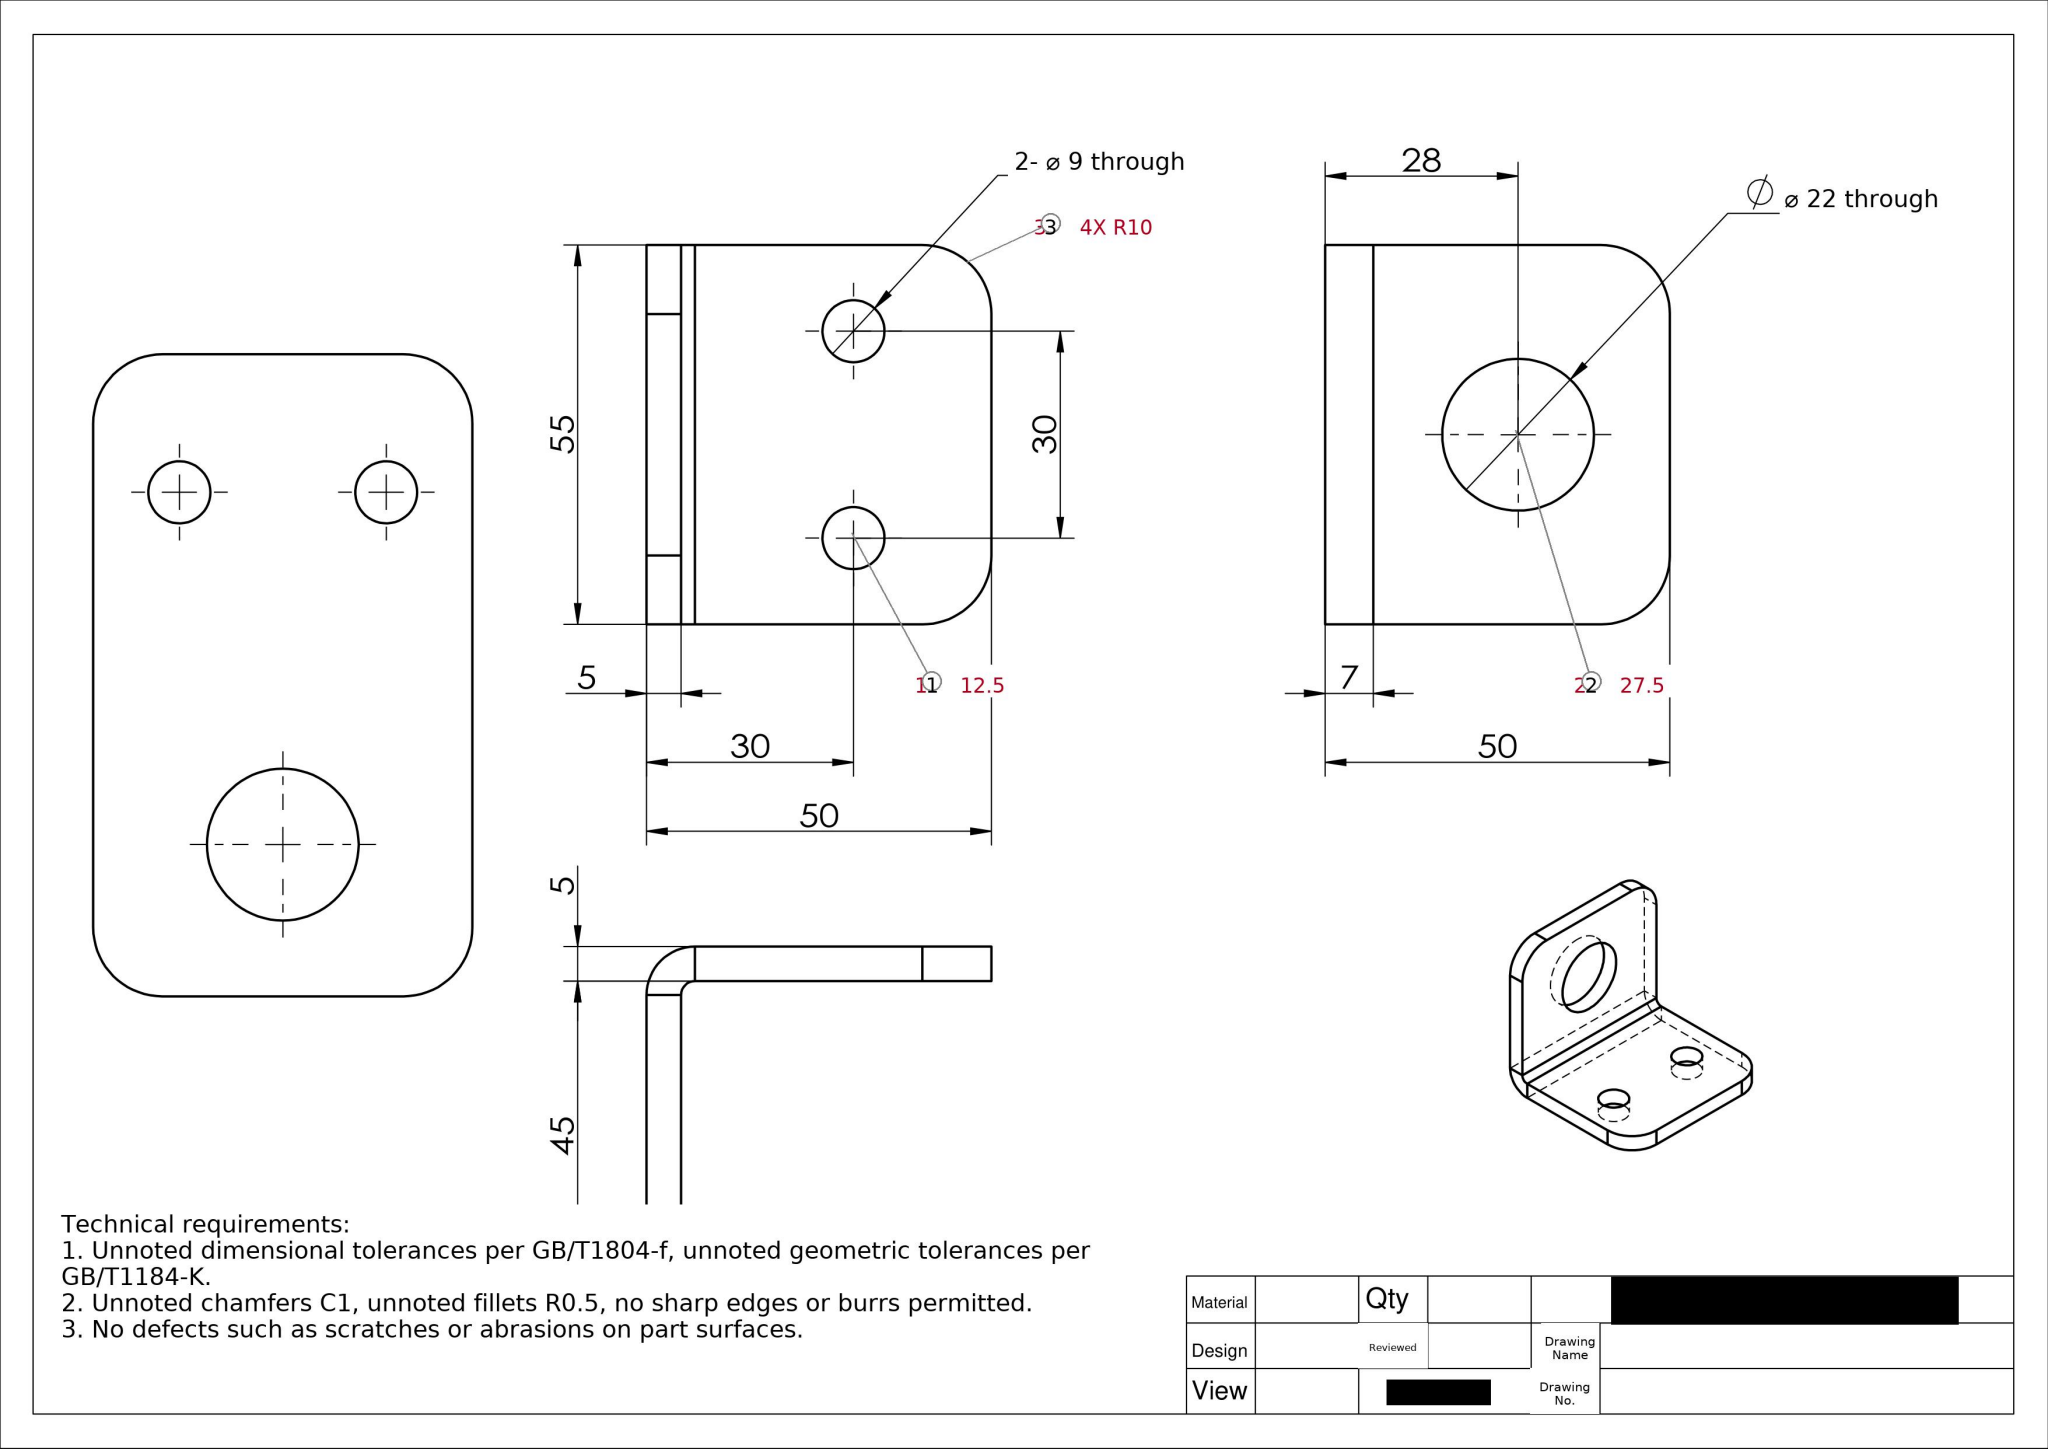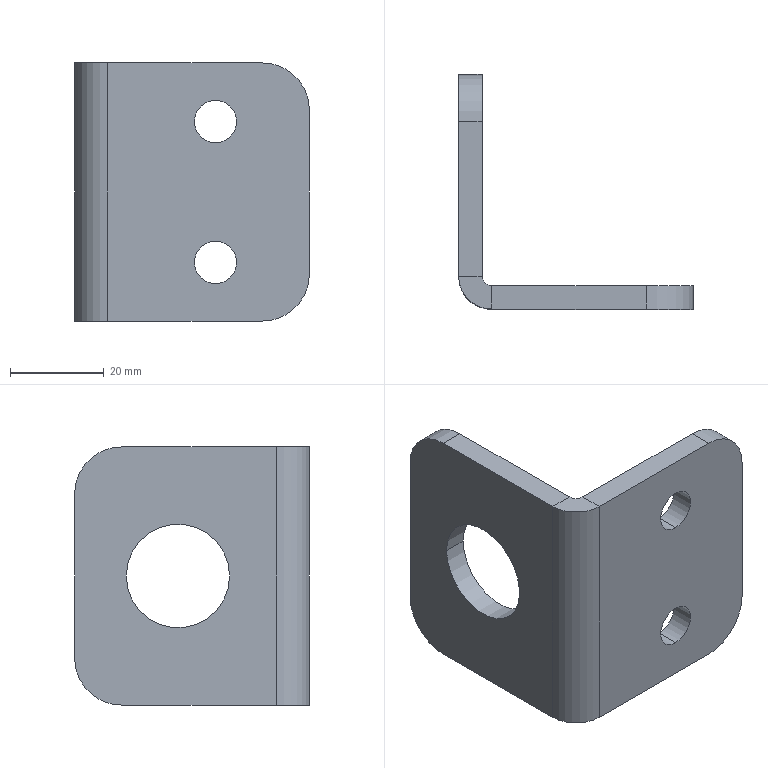Part | SolidWorks | mm | 1 solid | 24 faces | box 50 x 50 x 55 mm | volume 22628 mm3 | cylinder 12 | plane 12 | commonest cylinder face diameters 9 x4 20 x4 22 x2 4 x1 14 x1
STEP:
#1=CARTESIAN_POINT('',(30.,5.,38.));
#2=VERTEX_POINT('',#1);
#3=CARTESIAN_POINT('',(30.,5.,47.));
#4=VERTEX_POINT('',#3);
#5=CARTESIAN_POINT('',(30.,5.,42.5));
#6=DIRECTION('',(0.,1.,0.));
#7=DIRECTION('',(0.,0.,1.));
#8=AXIS2_PLACEMENT_3D('',#5,#6,#7);
#9=CIRCLE('',#8,4.5);
#10=EDGE_CURVE('',#2,#4,#9,.T.);
#11=ORIENTED_EDGE('',*,*,#10,.T.);
#12=CARTESIAN_POINT('',(30.,0.,47.));
#13=VERTEX_POINT('',#12);
#14=CARTESIAN_POINT('',(30.,10.,47.));
#15=DIRECTION('',(0.,-1.,0.));
#16=VECTOR('',#15,1000.);
#17=LINE('',#14,#16);
#18=EDGE_CURVE('',#4,#13,#17,.T.);
#19=ORIENTED_EDGE('',*,*,#18,.T.);
#20=CARTESIAN_POINT('',(30.,0.,38.));
#21=VERTEX_POINT('',#20);
#22=CARTESIAN_POINT('',(30.,0.,42.5));
#23=DIRECTION('',(0.,-1.,0.));
#24=DIRECTION('',(0.,0.,-1.));
#25=AXIS2_PLACEMENT_3D('',#22,#23,#24);
#26=CIRCLE('',#25,4.5);
#27=EDGE_CURVE('',#13,#21,#26,.T.);
#28=ORIENTED_EDGE('',*,*,#27,.T.);
#29=CARTESIAN_POINT('',(30.,10.,38.));
#30=DIRECTION('',(0.,-1.,0.));
#31=VECTOR('',#30,1000.);
#32=LINE('',#29,#31);
#33=EDGE_CURVE('',#2,#21,#32,.T.);
#34=ORIENTED_EDGE('',*,*,#33,.F.);
#35=EDGE_LOOP('',(#11,#19,#28,#34));
#36=FACE_OUTER_BOUND('',#35,.T.);
#37=CARTESIAN_POINT('',(30.,10.,42.5));
#38=DIRECTION('',(0.,-1.,0.));
#39=DIRECTION('',(0.,0.,-1.));
#40=AXIS2_PLACEMENT_3D('',#37,#38,#39);
#41=CYLINDRICAL_SURFACE('',#40,4.5);
#42=ADVANCED_FACE('',(#36),#41,.F.);
#43=CARTESIAN_POINT('',(30.,5.,8.));
#44=VERTEX_POINT('',#43);
#45=CARTESIAN_POINT('',(30.,5.,17.));
#46=VERTEX_POINT('',#45);
#47=CARTESIAN_POINT('',(30.,5.,12.5));
#48=DIRECTION('',(0.,1.,0.));
#49=DIRECTION('',(0.,0.,1.));
#50=AXIS2_PLACEMENT_3D('',#47,#48,#49);
#51=CIRCLE('',#50,4.5);
#52=EDGE_CURVE('',#44,#46,#51,.T.);
#53=ORIENTED_EDGE('',*,*,#52,.T.);
#54=CARTESIAN_POINT('',(30.,0.,17.));
#55=VERTEX_POINT('',#54);
#56=CARTESIAN_POINT('',(30.,10.,17.));
#57=DIRECTION('',(0.,-1.,0.));
#58=VECTOR('',#57,1000.);
#59=LINE('',#56,#58);
#60=EDGE_CURVE('',#46,#55,#59,.T.);
#61=ORIENTED_EDGE('',*,*,#60,.T.);
#62=CARTESIAN_POINT('',(30.,0.,8.));
#63=VERTEX_POINT('',#62);
#64=CARTESIAN_POINT('',(30.,0.,12.5));
#65=DIRECTION('',(0.,-1.,0.));
#66=DIRECTION('',(0.,0.,-1.));
#67=AXIS2_PLACEMENT_3D('',#64,#65,#66);
#68=CIRCLE('',#67,4.5);
#69=EDGE_CURVE('',#55,#63,#68,.T.);
#70=ORIENTED_EDGE('',*,*,#69,.T.);
#71=CARTESIAN_POINT('',(30.,10.,8.));
#72=DIRECTION('',(0.,-1.,0.));
#73=VECTOR('',#72,1000.);
#74=LINE('',#71,#73);
#75=EDGE_CURVE('',#44,#63,#74,.T.);
#76=ORIENTED_EDGE('',*,*,#75,.F.);
#77=EDGE_LOOP('',(#53,#61,#70,#76));
#78=FACE_OUTER_BOUND('',#77,.T.);
#79=CARTESIAN_POINT('',(30.,10.,12.5));
#80=DIRECTION('',(0.,-1.,0.));
#81=DIRECTION('',(0.,0.,-1.));
#82=AXIS2_PLACEMENT_3D('',#79,#80,#81);
#83=CYLINDRICAL_SURFACE('',#82,4.5);
#84=ADVANCED_FACE('',(#78),#83,.F.);
#85=CARTESIAN_POINT('',(0.,17.,27.5));
#86=VERTEX_POINT('',#85);
#87=CARTESIAN_POINT('',(0.,39.,27.5));
#88=VERTEX_POINT('',#87);
#89=CARTESIAN_POINT('',(0.,28.,27.5));
#90=DIRECTION('',(1.,-0.,0.));
#91=DIRECTION('',(0.,1.,0.));
#92=AXIS2_PLACEMENT_3D('',#89,#90,#91);
#93=CIRCLE('',#92,11.);
#94=EDGE_CURVE('',#86,#88,#93,.T.);
#95=ORIENTED_EDGE('',*,*,#94,.F.);
#96=CARTESIAN_POINT('',(5.,17.,27.5));
#97=VERTEX_POINT('',#96);
#98=CARTESIAN_POINT('',(5.,17.,27.5));
#99=DIRECTION('',(1.,-0.,0.));
#100=VECTOR('',#99,1000.);
#101=LINE('',#98,#100);
#102=EDGE_CURVE('',#86,#97,#101,.T.);
#103=ORIENTED_EDGE('',*,*,#102,.T.);
#104=CARTESIAN_POINT('',(5.,39.,27.5));
#105=VERTEX_POINT('',#104);
#106=CARTESIAN_POINT('',(5.,28.,27.5));
#107=DIRECTION('',(1.,-0.,0.));
#108=DIRECTION('',(0.,1.,0.));
#109=AXIS2_PLACEMENT_3D('',#106,#107,#108);
#110=CIRCLE('',#109,11.);
#111=EDGE_CURVE('',#97,#105,#110,.T.);
#112=ORIENTED_EDGE('',*,*,#111,.T.);
#113=CARTESIAN_POINT('',(5.,39.,27.5));
#114=DIRECTION('',(1.,-0.,0.));
#115=VECTOR('',#114,1000.);
#116=LINE('',#113,#115);
#117=EDGE_CURVE('',#88,#105,#116,.T.);
#118=ORIENTED_EDGE('',*,*,#117,.F.);
#119=EDGE_LOOP('',(#95,#103,#112,#118));
#120=FACE_OUTER_BOUND('',#119,.T.);
#121=CARTESIAN_POINT('',(5.,28.,27.5));
#122=DIRECTION('',(1.,-0.,0.));
#123=DIRECTION('',(0.,1.,0.));
#124=AXIS2_PLACEMENT_3D('',#121,#122,#123);
#125=CYLINDRICAL_SURFACE('',#124,11.);
#126=ADVANCED_FACE('',(#120),#125,.F.);
#127=CARTESIAN_POINT('',(0.,40.,0.));
#128=VERTEX_POINT('',#127);
#129=CARTESIAN_POINT('',(0.,7.,0.));
#130=VERTEX_POINT('',#129);
#131=CARTESIAN_POINT('',(0.,50.,0.));
#132=DIRECTION('',(-0.,-1.,0.));
#133=VECTOR('',#132,1000.);
#134=LINE('',#131,#133);
#135=EDGE_CURVE('',#128,#130,#134,.T.);
#136=ORIENTED_EDGE('',*,*,#135,.F.);
#137=CARTESIAN_POINT('',(5.,40.,0.));
#138=VERTEX_POINT('',#137);
#139=CARTESIAN_POINT('',(5.,40.,0.));
#140=DIRECTION('',(1.,-0.,0.));
#141=VECTOR('',#140,1000.);
#142=LINE('',#139,#141);
#143=EDGE_CURVE('',#128,#138,#142,.T.);
#144=ORIENTED_EDGE('',*,*,#143,.T.);
#145=CARTESIAN_POINT('',(5.,7.,0.));
#146=VERTEX_POINT('',#145);
#147=CARTESIAN_POINT('',(5.,50.,0.));
#148=DIRECTION('',(-0.,-1.,0.));
#149=VECTOR('',#148,1000.);
#150=LINE('',#147,#149);
#151=EDGE_CURVE('',#138,#146,#150,.T.);
#152=ORIENTED_EDGE('',*,*,#151,.T.);
#153=CARTESIAN_POINT('',(5.,7.,0.));
#154=DIRECTION('',(1.,-0.,0.));
#155=VECTOR('',#154,1000.);
#156=LINE('',#153,#155);
#157=EDGE_CURVE('',#130,#146,#156,.T.);
#158=ORIENTED_EDGE('',*,*,#157,.F.);
#159=EDGE_LOOP('',(#136,#144,#152,#158));
#160=FACE_OUTER_BOUND('',#159,.T.);
#161=CARTESIAN_POINT('',(5.,50.,0.));
#162=DIRECTION('',(0.,0.,1.));
#163=DIRECTION('',(-0.,-1.,0.));
#164=AXIS2_PLACEMENT_3D('',#161,#162,#163);
#165=PLANE('',#164);
#166=ADVANCED_FACE('',(#160),#165,.F.);
#167=CARTESIAN_POINT('',(5.,50.,45.));
#168=VERTEX_POINT('',#167);
#169=CARTESIAN_POINT('',(5.,50.,10.));
#170=VERTEX_POINT('',#169);
#171=CARTESIAN_POINT('',(5.,50.,55.));
#172=DIRECTION('',(0.,0.,-1.));
#173=VECTOR('',#172,1000.);
#174=LINE('',#171,#173);
#175=EDGE_CURVE('',#168,#170,#174,.T.);
#176=ORIENTED_EDGE('',*,*,#175,.T.);
#177=CARTESIAN_POINT('',(0.,50.,10.));
#178=VERTEX_POINT('',#177);
#179=CARTESIAN_POINT('',(5.,50.,10.));
#180=DIRECTION('',(-1.,0.,0.));
#181=VECTOR('',#180,1000.);
#182=LINE('',#179,#181);
#183=EDGE_CURVE('',#170,#178,#182,.T.);
#184=ORIENTED_EDGE('',*,*,#183,.T.);
#185=CARTESIAN_POINT('',(0.,50.,45.));
#186=VERTEX_POINT('',#185);
#187=CARTESIAN_POINT('',(0.,50.,55.));
#188=DIRECTION('',(0.,0.,-1.));
#189=VECTOR('',#188,1000.);
#190=LINE('',#187,#189);
#191=EDGE_CURVE('',#186,#178,#190,.T.);
#192=ORIENTED_EDGE('',*,*,#191,.F.);
#193=CARTESIAN_POINT('',(5.,50.,45.));
#194=DIRECTION('',(1.,-0.,0.));
#195=VECTOR('',#194,1000.);
#196=LINE('',#193,#195);
#197=EDGE_CURVE('',#186,#168,#196,.T.);
#198=ORIENTED_EDGE('',*,*,#197,.T.);
#199=EDGE_LOOP('',(#176,#184,#192,#198));
#200=FACE_OUTER_BOUND('',#199,.T.);
#201=CARTESIAN_POINT('',(5.,50.,55.));
#202=DIRECTION('',(-0.,-1.,0.));
#203=DIRECTION('',(0.,0.,-1.));
#204=AXIS2_PLACEMENT_3D('',#201,#202,#203);
#205=PLANE('',#204);
#206=ADVANCED_FACE('',(#200),#205,.F.);
#207=CARTESIAN_POINT('',(5.,40.,55.));
#208=VERTEX_POINT('',#207);
#209=CARTESIAN_POINT('',(5.,7.,55.));
#210=VERTEX_POINT('',#209);
#211=CARTESIAN_POINT('',(5.,50.,55.));
#212=DIRECTION('',(-0.,-1.,0.));
#213=VECTOR('',#212,1000.);
#214=LINE('',#211,#213);
#215=EDGE_CURVE('',#208,#210,#214,.T.);
#216=ORIENTED_EDGE('',*,*,#215,.F.);
#217=CARTESIAN_POINT('',(0.,40.,55.));
#218=VERTEX_POINT('',#217);
#219=CARTESIAN_POINT('',(5.,40.,55.));
#220=DIRECTION('',(-1.,0.,0.));
#221=VECTOR('',#220,1000.);
#222=LINE('',#219,#221);
#223=EDGE_CURVE('',#208,#218,#222,.T.);
#224=ORIENTED_EDGE('',*,*,#223,.T.);
#225=CARTESIAN_POINT('',(-0.,7.,55.));
#226=VERTEX_POINT('',#225);
#227=CARTESIAN_POINT('',(0.,50.,55.));
#228=DIRECTION('',(-0.,-1.,0.));
#229=VECTOR('',#228,1000.);
#230=LINE('',#227,#229);
#231=EDGE_CURVE('',#218,#226,#230,.T.);
#232=ORIENTED_EDGE('',*,*,#231,.T.);
#233=CARTESIAN_POINT('',(5.,7.,55.));
#234=DIRECTION('',(1.,0.,0.));
#235=VECTOR('',#234,1000.);
#236=LINE('',#233,#235);
#237=EDGE_CURVE('',#226,#210,#236,.T.);
#238=ORIENTED_EDGE('',*,*,#237,.T.);
#239=EDGE_LOOP('',(#216,#224,#232,#238));
#240=FACE_OUTER_BOUND('',#239,.T.);
#241=CARTESIAN_POINT('',(5.,50.,55.));
#242=DIRECTION('',(0.,0.,1.));
#243=DIRECTION('',(-0.,-1.,0.));
#244=AXIS2_PLACEMENT_3D('',#241,#242,#243);
#245=PLANE('',#244);
#246=ADVANCED_FACE('',(#240),#245,.T.);
#247=ORIENTED_EDGE('',*,*,#237,.F.);
#248=CARTESIAN_POINT('',(7.,-0.,55.));
#249=VERTEX_POINT('',#248);
#250=CARTESIAN_POINT('',(7.,7.,55.));
#251=DIRECTION('',(0.,0.,1.));
#252=DIRECTION('',(1.,0.,0.));
#253=AXIS2_PLACEMENT_3D('',#250,#251,#252);
#254=CIRCLE('',#253,7.);
#255=EDGE_CURVE('',#226,#249,#254,.T.);
#256=ORIENTED_EDGE('',*,*,#255,.T.);
#257=CARTESIAN_POINT('',(7.,5.,55.));
#258=VERTEX_POINT('',#257);
#259=CARTESIAN_POINT('',(7.,5.,55.));
#260=DIRECTION('',(0.,1.,0.));
#261=VECTOR('',#260,1000.);
#262=LINE('',#259,#261);
#263=EDGE_CURVE('',#249,#258,#262,.T.);
#264=ORIENTED_EDGE('',*,*,#263,.T.);
#265=CARTESIAN_POINT('',(7.,7.,55.));
#266=DIRECTION('',(0.,0.,1.));
#267=DIRECTION('',(-1.,0.,0.));
#268=AXIS2_PLACEMENT_3D('',#265,#266,#267);
#269=CIRCLE('',#268,2.);
#270=EDGE_CURVE('',#210,#258,#269,.T.);
#271=ORIENTED_EDGE('',*,*,#270,.F.);
#272=EDGE_LOOP('',(#247,#256,#264,#271));
#273=FACE_OUTER_BOUND('',#272,.T.);
#274=CARTESIAN_POINT('',(7.,7.,55.));
#275=DIRECTION('',(0.,0.,1.));
#276=DIRECTION('',(1.,0.,0.));
#277=AXIS2_PLACEMENT_3D('',#274,#275,#276);
#278=PLANE('',#277);
#279=ADVANCED_FACE('',(#273),#278,.T.);
#280=CARTESIAN_POINT('',(40.,0.,55.));
#281=VERTEX_POINT('',#280);
#282=CARTESIAN_POINT('',(0.,0.,55.));
#283=DIRECTION('',(1.,0.,0.));
#284=VECTOR('',#283,1000.);
#285=LINE('',#282,#284);
#286=EDGE_CURVE('',#249,#281,#285,.T.);
#287=ORIENTED_EDGE('',*,*,#286,.T.);
#288=CARTESIAN_POINT('',(40.,5.,55.));
#289=VERTEX_POINT('',#288);
#290=CARTESIAN_POINT('',(40.,5.,55.));
#291=DIRECTION('',(0.,1.,0.));
#292=VECTOR('',#291,1000.);
#293=LINE('',#290,#292);
#294=EDGE_CURVE('',#281,#289,#293,.T.);
#295=ORIENTED_EDGE('',*,*,#294,.T.);
#296=CARTESIAN_POINT('',(0.,5.,55.));
#297=DIRECTION('',(1.,0.,0.));
#298=VECTOR('',#297,1000.);
#299=LINE('',#296,#298);
#300=EDGE_CURVE('',#258,#289,#299,.T.);
#301=ORIENTED_EDGE('',*,*,#300,.F.);
#302=ORIENTED_EDGE('',*,*,#263,.F.);
#303=EDGE_LOOP('',(#287,#295,#301,#302));
#304=FACE_OUTER_BOUND('',#303,.T.);
#305=CARTESIAN_POINT('',(0.,5.,55.));
#306=DIRECTION('',(0.,0.,1.));
#307=DIRECTION('',(1.,0.,0.));
#308=AXIS2_PLACEMENT_3D('',#305,#306,#307);
#309=PLANE('',#308);
#310=ADVANCED_FACE('',(#304),#309,.T.);
#311=CARTESIAN_POINT('',(50.,5.,45.));
#312=VERTEX_POINT('',#311);
#313=CARTESIAN_POINT('',(50.,5.,10.));
#314=VERTEX_POINT('',#313);
#315=CARTESIAN_POINT('',(50.,5.,55.));
#316=DIRECTION('',(0.,0.,-1.));
#317=VECTOR('',#316,1000.);
#318=LINE('',#315,#317);
#319=EDGE_CURVE('',#312,#314,#318,.T.);
#320=ORIENTED_EDGE('',*,*,#319,.F.);
#321=CARTESIAN_POINT('',(50.,0.,45.));
#322=VERTEX_POINT('',#321);
#323=CARTESIAN_POINT('',(50.,5.,45.));
#324=DIRECTION('',(0.,-1.,0.));
#325=VECTOR('',#324,1000.);
#326=LINE('',#323,#325);
#327=EDGE_CURVE('',#312,#322,#326,.T.);
#328=ORIENTED_EDGE('',*,*,#327,.T.);
#329=CARTESIAN_POINT('',(50.,0.,10.));
#330=VERTEX_POINT('',#329);
#331=CARTESIAN_POINT('',(50.,0.,55.));
#332=DIRECTION('',(0.,0.,-1.));
#333=VECTOR('',#332,1000.);
#334=LINE('',#331,#333);
#335=EDGE_CURVE('',#322,#330,#334,.T.);
#336=ORIENTED_EDGE('',*,*,#335,.T.);
#337=CARTESIAN_POINT('',(50.,5.,10.));
#338=DIRECTION('',(0.,1.,0.));
#339=VECTOR('',#338,1000.);
#340=LINE('',#337,#339);
#341=EDGE_CURVE('',#330,#314,#340,.T.);
#342=ORIENTED_EDGE('',*,*,#341,.T.);
#343=EDGE_LOOP('',(#320,#328,#336,#342));
#344=FACE_OUTER_BOUND('',#343,.T.);
#345=CARTESIAN_POINT('',(50.,5.,55.));
#346=DIRECTION('',(1.,0.,0.));
#347=DIRECTION('',(0.,0.,-1.));
#348=AXIS2_PLACEMENT_3D('',#345,#346,#347);
#349=PLANE('',#348);
#350=ADVANCED_FACE('',(#344),#349,.T.);
#351=CARTESIAN_POINT('',(7.,5.,0.));
#352=VERTEX_POINT('',#351);
#353=CARTESIAN_POINT('',(40.,5.,0.));
#354=VERTEX_POINT('',#353);
#355=CARTESIAN_POINT('',(0.,5.,0.));
#356=DIRECTION('',(1.,0.,0.));
#357=VECTOR('',#356,1000.);
#358=LINE('',#355,#357);
#359=EDGE_CURVE('',#352,#354,#358,.T.);
#360=ORIENTED_EDGE('',*,*,#359,.T.);
#361=CARTESIAN_POINT('',(40.,0.,0.));
#362=VERTEX_POINT('',#361);
#363=CARTESIAN_POINT('',(40.,5.,0.));
#364=DIRECTION('',(0.,-1.,0.));
#365=VECTOR('',#364,1000.);
#366=LINE('',#363,#365);
#367=EDGE_CURVE('',#354,#362,#366,.T.);
#368=ORIENTED_EDGE('',*,*,#367,.T.);
#369=CARTESIAN_POINT('',(7.,0.,0.));
#370=VERTEX_POINT('',#369);
#371=CARTESIAN_POINT('',(0.,0.,0.));
#372=DIRECTION('',(1.,0.,0.));
#373=VECTOR('',#372,1000.);
#374=LINE('',#371,#373);
#375=EDGE_CURVE('',#370,#362,#374,.T.);
#376=ORIENTED_EDGE('',*,*,#375,.F.);
#377=CARTESIAN_POINT('',(7.,5.,0.));
#378=DIRECTION('',(0.,1.,0.));
#379=VECTOR('',#378,1000.);
#380=LINE('',#377,#379);
#381=EDGE_CURVE('',#370,#352,#380,.T.);
#382=ORIENTED_EDGE('',*,*,#381,.T.);
#383=EDGE_LOOP('',(#360,#368,#376,#382));
#384=FACE_OUTER_BOUND('',#383,.T.);
#385=CARTESIAN_POINT('',(0.,5.,0.));
#386=DIRECTION('',(0.,0.,1.));
#387=DIRECTION('',(1.,0.,0.));
#388=AXIS2_PLACEMENT_3D('',#385,#386,#387);
#389=PLANE('',#388);
#390=ADVANCED_FACE('',(#384),#389,.F.);
#391=ORIENTED_EDGE('',*,*,#102,.F.);
#392=CARTESIAN_POINT('',(0.,28.,27.5));
#393=DIRECTION('',(1.,-0.,0.));
#394=DIRECTION('',(0.,1.,0.));
#395=AXIS2_PLACEMENT_3D('',#392,#393,#394);
#396=CIRCLE('',#395,11.);
#397=EDGE_CURVE('',#88,#86,#396,.T.);
#398=ORIENTED_EDGE('',*,*,#397,.F.);
#399=ORIENTED_EDGE('',*,*,#117,.T.);
#400=CARTESIAN_POINT('',(5.,28.,27.5));
#401=DIRECTION('',(1.,-0.,0.));
#402=DIRECTION('',(0.,1.,0.));
#403=AXIS2_PLACEMENT_3D('',#400,#401,#402);
#404=CIRCLE('',#403,11.);
#405=EDGE_CURVE('',#105,#97,#404,.T.);
#406=ORIENTED_EDGE('',*,*,#405,.T.);
#407=EDGE_LOOP('',(#391,#398,#399,#406));
#408=FACE_OUTER_BOUND('',#407,.T.);
#409=CARTESIAN_POINT('',(5.,28.,27.5));
#410=DIRECTION('',(1.,-0.,0.));
#411=DIRECTION('',(0.,1.,0.));
#412=AXIS2_PLACEMENT_3D('',#409,#410,#411);
#413=CYLINDRICAL_SURFACE('',#412,11.);
#414=ADVANCED_FACE('',(#408),#413,.F.);
#415=CARTESIAN_POINT('',(7.,7.,0.));
#416=DIRECTION('',(0.,0.,-1.));
#417=DIRECTION('',(1.,0.,0.));
#418=AXIS2_PLACEMENT_3D('',#415,#416,#417);
#419=CIRCLE('',#418,7.);
#420=EDGE_CURVE('',#370,#130,#419,.T.);
#421=ORIENTED_EDGE('',*,*,#420,.T.);
#422=ORIENTED_EDGE('',*,*,#157,.T.);
#423=CARTESIAN_POINT('',(7.,7.,0.));
#424=DIRECTION('',(0.,0.,-1.));
#425=DIRECTION('',(1.,0.,0.));
#426=AXIS2_PLACEMENT_3D('',#423,#424,#425);
#427=CIRCLE('',#426,2.);
#428=EDGE_CURVE('',#352,#146,#427,.T.);
#429=ORIENTED_EDGE('',*,*,#428,.F.);
#430=ORIENTED_EDGE('',*,*,#381,.F.);
#431=EDGE_LOOP('',(#421,#422,#429,#430));
#432=FACE_OUTER_BOUND('',#431,.T.);
#433=CARTESIAN_POINT('',(7.,7.,0.));
#434=DIRECTION('',(0.,0.,-1.));
#435=DIRECTION('',(-1.,0.,0.));
#436=AXIS2_PLACEMENT_3D('',#433,#434,#435);
#437=PLANE('',#436);
#438=ADVANCED_FACE('',(#432),#437,.T.);
#439=ORIENTED_EDGE('',*,*,#10,.F.);
#440=CARTESIAN_POINT('',(30.,5.,42.5));
#441=DIRECTION('',(0.,1.,0.));
#442=DIRECTION('',(0.,0.,1.));
#443=AXIS2_PLACEMENT_3D('',#440,#441,#442);
#444=CIRCLE('',#443,4.5);
#445=EDGE_CURVE('',#4,#2,#444,.T.);
#446=ORIENTED_EDGE('',*,*,#445,.F.);
#447=EDGE_LOOP('',(#439,#446));
#448=FACE_BOUND('',#447,.T.);
#449=ORIENTED_EDGE('',*,*,#52,.F.);
#450=CARTESIAN_POINT('',(30.,5.,12.5));
#451=DIRECTION('',(0.,1.,0.));
#452=DIRECTION('',(0.,0.,1.));
#453=AXIS2_PLACEMENT_3D('',#450,#451,#452);
#454=CIRCLE('',#453,4.5);
#455=EDGE_CURVE('',#46,#44,#454,.T.);
#456=ORIENTED_EDGE('',*,*,#455,.F.);
#457=EDGE_LOOP('',(#449,#456));
#458=FACE_BOUND('',#457,.T.);
#459=ORIENTED_EDGE('',*,*,#300,.T.);
#460=CARTESIAN_POINT('',(40.,5.,45.));
#461=DIRECTION('',(0.,1.,0.));
#462=DIRECTION('',(0.,0.,1.));
#463=AXIS2_PLACEMENT_3D('',#460,#461,#462);
#464=CIRCLE('',#463,10.);
#465=EDGE_CURVE('',#289,#312,#464,.T.);
#466=ORIENTED_EDGE('',*,*,#465,.T.);
#467=ORIENTED_EDGE('',*,*,#319,.T.);
#468=CARTESIAN_POINT('',(40.,5.,10.));
#469=DIRECTION('',(0.,1.,0.));
#470=DIRECTION('',(0.,0.,1.));
#471=AXIS2_PLACEMENT_3D('',#468,#469,#470);
#472=CIRCLE('',#471,10.);
#473=EDGE_CURVE('',#314,#354,#472,.T.);
#474=ORIENTED_EDGE('',*,*,#473,.T.);
#475=ORIENTED_EDGE('',*,*,#359,.F.);
#476=CARTESIAN_POINT('',(7.,5.,55.));
#477=DIRECTION('',(0.,0.,1.));
#478=VECTOR('',#477,1000.);
#479=LINE('',#476,#478);
#480=EDGE_CURVE('',#352,#258,#479,.T.);
#481=ORIENTED_EDGE('',*,*,#480,.T.);
#482=EDGE_LOOP('',(#459,#466,#467,#474,#475,#481));
#483=FACE_OUTER_BOUND('',#482,.T.);
#484=CARTESIAN_POINT('',(0.,5.,55.));
#485=DIRECTION('',(0.,1.,0.));
#486=DIRECTION('',(0.,0.,1.));
#487=AXIS2_PLACEMENT_3D('',#484,#485,#486);
#488=PLANE('',#487);
#489=ADVANCED_FACE('',(#448,#458,#483),#488,.T.);
#490=ORIENTED_EDGE('',*,*,#405,.F.);
#491=ORIENTED_EDGE('',*,*,#111,.F.);
#492=EDGE_LOOP('',(#490,#491));
#493=FACE_BOUND('',#492,.T.);
#494=ORIENTED_EDGE('',*,*,#151,.F.);
#495=CARTESIAN_POINT('',(5.,40.,10.));
#496=DIRECTION('',(1.,-0.,0.));
#497=DIRECTION('',(0.,1.,0.));
#498=AXIS2_PLACEMENT_3D('',#495,#496,#497);
#499=CIRCLE('',#498,10.);
#500=EDGE_CURVE('',#138,#170,#499,.T.);
#501=ORIENTED_EDGE('',*,*,#500,.T.);
#502=ORIENTED_EDGE('',*,*,#175,.F.);
#503=CARTESIAN_POINT('',(5.,40.,45.));
#504=DIRECTION('',(1.,-0.,0.));
#505=DIRECTION('',(0.,1.,0.));
#506=AXIS2_PLACEMENT_3D('',#503,#504,#505);
#507=CIRCLE('',#506,10.);
#508=EDGE_CURVE('',#168,#208,#507,.T.);
#509=ORIENTED_EDGE('',*,*,#508,.T.);
#510=ORIENTED_EDGE('',*,*,#215,.T.);
#511=CARTESIAN_POINT('',(5.,7.,0.));
#512=DIRECTION('',(0.,0.,-1.));
#513=VECTOR('',#512,1000.);
#514=LINE('',#511,#513);
#515=EDGE_CURVE('',#210,#146,#514,.T.);
#516=ORIENTED_EDGE('',*,*,#515,.T.);
#517=EDGE_LOOP('',(#494,#501,#502,#509,#510,#516));
#518=FACE_OUTER_BOUND('',#517,.T.);
#519=CARTESIAN_POINT('',(5.,50.,55.));
#520=DIRECTION('',(1.,-0.,0.));
#521=DIRECTION('',(0.,1.,0.));
#522=AXIS2_PLACEMENT_3D('',#519,#520,#521);
#523=PLANE('',#522);
#524=ADVANCED_FACE('',(#493,#518),#523,.T.);
#525=ORIENTED_EDGE('',*,*,#270,.T.);
#526=ORIENTED_EDGE('',*,*,#480,.F.);
#527=ORIENTED_EDGE('',*,*,#428,.T.);
#528=ORIENTED_EDGE('',*,*,#515,.F.);
#529=EDGE_LOOP('',(#525,#526,#527,#528));
#530=FACE_OUTER_BOUND('',#529,.T.);
#531=CARTESIAN_POINT('',(7.,7.,55.));
#532=DIRECTION('',(0.,0.,1.));
#533=DIRECTION('',(1.,0.,0.));
#534=AXIS2_PLACEMENT_3D('',#531,#532,#533);
#535=CYLINDRICAL_SURFACE('',#534,2.);
#536=ADVANCED_FACE('',(#530),#535,.F.);
#537=CARTESIAN_POINT('',(30.,0.,42.5));
#538=DIRECTION('',(0.,-1.,0.));
#539=DIRECTION('',(0.,0.,-1.));
#540=AXIS2_PLACEMENT_3D('',#537,#538,#539);
#541=CIRCLE('',#540,4.5);
#542=EDGE_CURVE('',#21,#13,#541,.T.);
#543=ORIENTED_EDGE('',*,*,#542,.F.);
#544=ORIENTED_EDGE('',*,*,#27,.F.);
#545=EDGE_LOOP('',(#543,#544));
#546=FACE_BOUND('',#545,.T.);
#547=CARTESIAN_POINT('',(30.,0.,12.5));
#548=DIRECTION('',(0.,-1.,0.));
#549=DIRECTION('',(0.,0.,-1.));
#550=AXIS2_PLACEMENT_3D('',#547,#548,#549);
#551=CIRCLE('',#550,4.5);
#552=EDGE_CURVE('',#63,#55,#551,.T.);
#553=ORIENTED_EDGE('',*,*,#552,.F.);
#554=ORIENTED_EDGE('',*,*,#69,.F.);
#555=EDGE_LOOP('',(#553,#554));
#556=FACE_BOUND('',#555,.T.);
#557=ORIENTED_EDGE('',*,*,#335,.F.);
#558=CARTESIAN_POINT('',(40.,0.,45.));
#559=DIRECTION('',(0.,-1.,0.));
#560=DIRECTION('',(0.,0.,1.));
#561=AXIS2_PLACEMENT_3D('',#558,#559,#560);
#562=CIRCLE('',#561,10.);
#563=EDGE_CURVE('',#322,#281,#562,.T.);
#564=ORIENTED_EDGE('',*,*,#563,.T.);
#565=ORIENTED_EDGE('',*,*,#286,.F.);
#566=CARTESIAN_POINT('',(7.,0.,55.));
#567=DIRECTION('',(0.,0.,1.));
#568=VECTOR('',#567,1000.);
#569=LINE('',#566,#568);
#570=EDGE_CURVE('',#370,#249,#569,.T.);
#571=ORIENTED_EDGE('',*,*,#570,.F.);
#572=ORIENTED_EDGE('',*,*,#375,.T.);
#573=CARTESIAN_POINT('',(40.,0.,10.));
#574=DIRECTION('',(0.,-1.,0.));
#575=DIRECTION('',(0.,0.,1.));
#576=AXIS2_PLACEMENT_3D('',#573,#574,#575);
#577=CIRCLE('',#576,10.);
#578=EDGE_CURVE('',#362,#330,#577,.T.);
#579=ORIENTED_EDGE('',*,*,#578,.T.);
#580=EDGE_LOOP('',(#557,#564,#565,#571,#572,#579));
#581=FACE_OUTER_BOUND('',#580,.T.);
#582=CARTESIAN_POINT('',(0.,0.,55.));
#583=DIRECTION('',(0.,1.,0.));
#584=DIRECTION('',(0.,0.,1.));
#585=AXIS2_PLACEMENT_3D('',#582,#583,#584);
#586=PLANE('',#585);
#587=ADVANCED_FACE('',(#546,#556,#581),#586,.F.);
#588=ORIENTED_EDGE('',*,*,#397,.T.);
#589=ORIENTED_EDGE('',*,*,#94,.T.);
#590=EDGE_LOOP('',(#588,#589));
#591=FACE_BOUND('',#590,.T.);
#592=ORIENTED_EDGE('',*,*,#191,.T.);
#593=CARTESIAN_POINT('',(0.,40.,10.));
#594=DIRECTION('',(-1.,0.,0.));
#595=DIRECTION('',(0.,1.,0.));
#596=AXIS2_PLACEMENT_3D('',#593,#594,#595);
#597=CIRCLE('',#596,10.);
#598=EDGE_CURVE('',#178,#128,#597,.T.);
#599=ORIENTED_EDGE('',*,*,#598,.T.);
#600=ORIENTED_EDGE('',*,*,#135,.T.);
#601=CARTESIAN_POINT('',(-0.,7.,55.));
#602=DIRECTION('',(0.,0.,-1.));
#603=VECTOR('',#602,1000.);
#604=LINE('',#601,#603);
#605=EDGE_CURVE('',#226,#130,#604,.T.);
#606=ORIENTED_EDGE('',*,*,#605,.F.);
#607=ORIENTED_EDGE('',*,*,#231,.F.);
#608=CARTESIAN_POINT('',(0.,40.,45.));
#609=DIRECTION('',(-1.,0.,0.));
#610=DIRECTION('',(0.,1.,0.));
#611=AXIS2_PLACEMENT_3D('',#608,#609,#610);
#612=CIRCLE('',#611,10.);
#613=EDGE_CURVE('',#218,#186,#612,.T.);
#614=ORIENTED_EDGE('',*,*,#613,.T.);
#615=EDGE_LOOP('',(#592,#599,#600,#606,#607,#614));
#616=FACE_OUTER_BOUND('',#615,.T.);
#617=CARTESIAN_POINT('',(0.,50.,55.));
#618=DIRECTION('',(1.,-0.,0.));
#619=DIRECTION('',(0.,1.,0.));
#620=AXIS2_PLACEMENT_3D('',#617,#618,#619);
#621=PLANE('',#620);
#622=ADVANCED_FACE('',(#591,#616),#621,.F.);
#623=ORIENTED_EDGE('',*,*,#255,.F.);
#624=ORIENTED_EDGE('',*,*,#605,.T.);
#625=ORIENTED_EDGE('',*,*,#420,.F.);
#626=ORIENTED_EDGE('',*,*,#570,.T.);
#627=EDGE_LOOP('',(#623,#624,#625,#626));
#628=FACE_OUTER_BOUND('',#627,.T.);
#629=CARTESIAN_POINT('',(7.,7.,55.));
#630=DIRECTION('',(0.,0.,1.));
#631=DIRECTION('',(1.,0.,0.));
#632=AXIS2_PLACEMENT_3D('',#629,#630,#631);
#633=CYLINDRICAL_SURFACE('',#632,7.);
#634=ADVANCED_FACE('',(#628),#633,.T.);
#635=ORIENTED_EDGE('',*,*,#60,.F.);
#636=ORIENTED_EDGE('',*,*,#455,.T.);
#637=ORIENTED_EDGE('',*,*,#75,.T.);
#638=ORIENTED_EDGE('',*,*,#552,.T.);
#639=EDGE_LOOP('',(#635,#636,#637,#638));
#640=FACE_OUTER_BOUND('',#639,.T.);
#641=CARTESIAN_POINT('',(30.,10.,12.5));
#642=DIRECTION('',(0.,-1.,0.));
#643=DIRECTION('',(0.,0.,-1.));
#644=AXIS2_PLACEMENT_3D('',#641,#642,#643);
#645=CYLINDRICAL_SURFACE('',#644,4.5);
#646=ADVANCED_FACE('',(#640),#645,.F.);
#647=ORIENTED_EDGE('',*,*,#18,.F.);
#648=ORIENTED_EDGE('',*,*,#445,.T.);
#649=ORIENTED_EDGE('',*,*,#33,.T.);
#650=ORIENTED_EDGE('',*,*,#542,.T.);
#651=EDGE_LOOP('',(#647,#648,#649,#650));
#652=FACE_OUTER_BOUND('',#651,.T.);
#653=CARTESIAN_POINT('',(30.,10.,42.5));
#654=DIRECTION('',(0.,-1.,0.));
#655=DIRECTION('',(0.,0.,-1.));
#656=AXIS2_PLACEMENT_3D('',#653,#654,#655);
#657=CYLINDRICAL_SURFACE('',#656,4.5);
#658=ADVANCED_FACE('',(#652),#657,.F.);
#659=ORIENTED_EDGE('',*,*,#563,.F.);
#660=ORIENTED_EDGE('',*,*,#327,.F.);
#661=ORIENTED_EDGE('',*,*,#465,.F.);
#662=ORIENTED_EDGE('',*,*,#294,.F.);
#663=EDGE_LOOP('',(#659,#660,#661,#662));
#664=FACE_OUTER_BOUND('',#663,.T.);
#665=CARTESIAN_POINT('',(40.,5.,45.));
#666=DIRECTION('',(0.,1.,0.));
#667=DIRECTION('',(0.,0.,1.));
#668=AXIS2_PLACEMENT_3D('',#665,#666,#667);
#669=CYLINDRICAL_SURFACE('',#668,10.);
#670=ADVANCED_FACE('',(#664),#669,.T.);
#671=ORIENTED_EDGE('',*,*,#578,.F.);
#672=ORIENTED_EDGE('',*,*,#367,.F.);
#673=ORIENTED_EDGE('',*,*,#473,.F.);
#674=ORIENTED_EDGE('',*,*,#341,.F.);
#675=EDGE_LOOP('',(#671,#672,#673,#674));
#676=FACE_OUTER_BOUND('',#675,.T.);
#677=CARTESIAN_POINT('',(40.,5.,10.));
#678=DIRECTION('',(0.,-1.,0.));
#679=DIRECTION('',(0.,0.,-1.));
#680=AXIS2_PLACEMENT_3D('',#677,#678,#679);
#681=CYLINDRICAL_SURFACE('',#680,10.);
#682=ADVANCED_FACE('',(#676),#681,.T.);
#683=ORIENTED_EDGE('',*,*,#598,.F.);
#684=ORIENTED_EDGE('',*,*,#183,.F.);
#685=ORIENTED_EDGE('',*,*,#500,.F.);
#686=ORIENTED_EDGE('',*,*,#143,.F.);
#687=EDGE_LOOP('',(#683,#684,#685,#686));
#688=FACE_OUTER_BOUND('',#687,.T.);
#689=CARTESIAN_POINT('',(5.,40.,10.));
#690=DIRECTION('',(1.,-0.,0.));
#691=DIRECTION('',(0.,1.,0.));
#692=AXIS2_PLACEMENT_3D('',#689,#690,#691);
#693=CYLINDRICAL_SURFACE('',#692,10.);
#694=ADVANCED_FACE('',(#688),#693,.T.);
#695=ORIENTED_EDGE('',*,*,#613,.F.);
#696=ORIENTED_EDGE('',*,*,#223,.F.);
#697=ORIENTED_EDGE('',*,*,#508,.F.);
#698=ORIENTED_EDGE('',*,*,#197,.F.);
#699=EDGE_LOOP('',(#695,#696,#697,#698));
#700=FACE_OUTER_BOUND('',#699,.T.);
#701=CARTESIAN_POINT('',(5.,40.,45.));
#702=DIRECTION('',(-1.,0.,0.));
#703=DIRECTION('',(0.,-1.,0.));
#704=AXIS2_PLACEMENT_3D('',#701,#702,#703);
#705=CYLINDRICAL_SURFACE('',#704,10.);
#706=ADVANCED_FACE('',(#700),#705,.T.);
#707=CLOSED_SHELL('',(#42,#84,#126,#166,#206,#246,#279,#310,#350,#390,#414,#438,#489,#524,#536,#587,#622,#634,#646,#658,#670,#682,#694,#706));
#708=MANIFOLD_SOLID_BREP('',#707);
#709=CARTESIAN_POINT('',(0.,0.,0.));
#710=DIRECTION('',(0.,0.,1.));
#711=DIRECTION('',(1.,0.,0.));
#712=AXIS2_PLACEMENT_3D('',#709,#710,#711);
#713=(LENGTH_UNIT()NAMED_UNIT(*)SI_UNIT(.MILLI.,.METRE.));
#714=UNCERTAINTY_MEASURE_WITH_UNIT(LENGTH_MEASURE(0.00001),#713,'','');
#715=(NAMED_UNIT(*)PLANE_ANGLE_UNIT()SI_UNIT($,.RADIAN.));
#716=(NAMED_UNIT(*)SI_UNIT($,.STERADIAN.)SOLID_ANGLE_UNIT());
#717=(GEOMETRIC_REPRESENTATION_CONTEXT(3)GLOBAL_UNCERTAINTY_ASSIGNED_CONTEXT((#714))GLOBAL_UNIT_ASSIGNED_CONTEXT((#713,#715,#716))REPRESENTATION_CONTEXT('',''));
#718=ADVANCED_BREP_SHAPE_REPRESENTATION('',(#708,#712),#717);